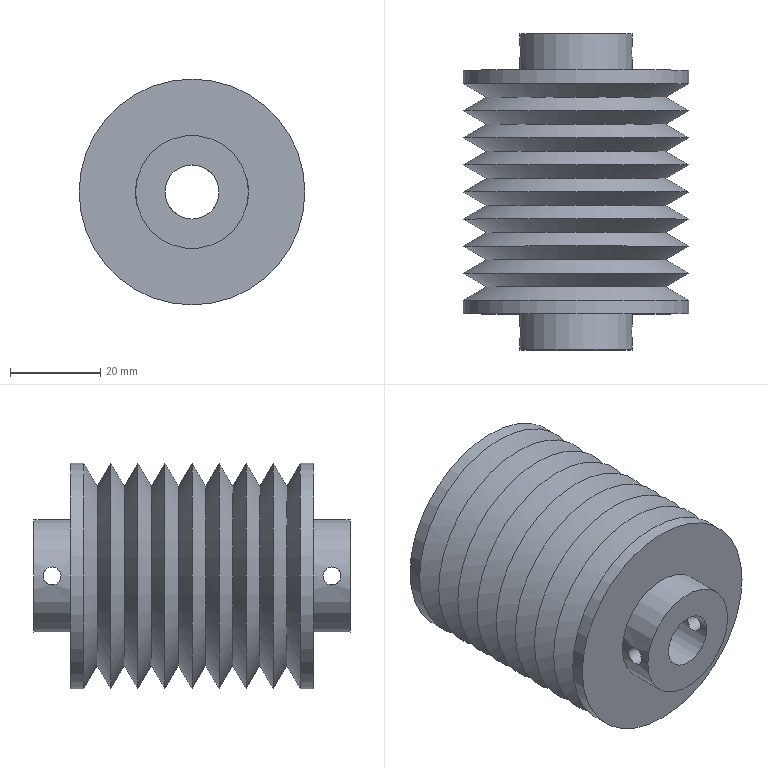Component | NX | SMALL_PULLEY | 1 solid | 29 faces | volume 87405 mm3 | cone 16 | cylinder 9 | plane 4 | commonest cylinder face diameters 4 x4 25 x2 50 x2 12 x1